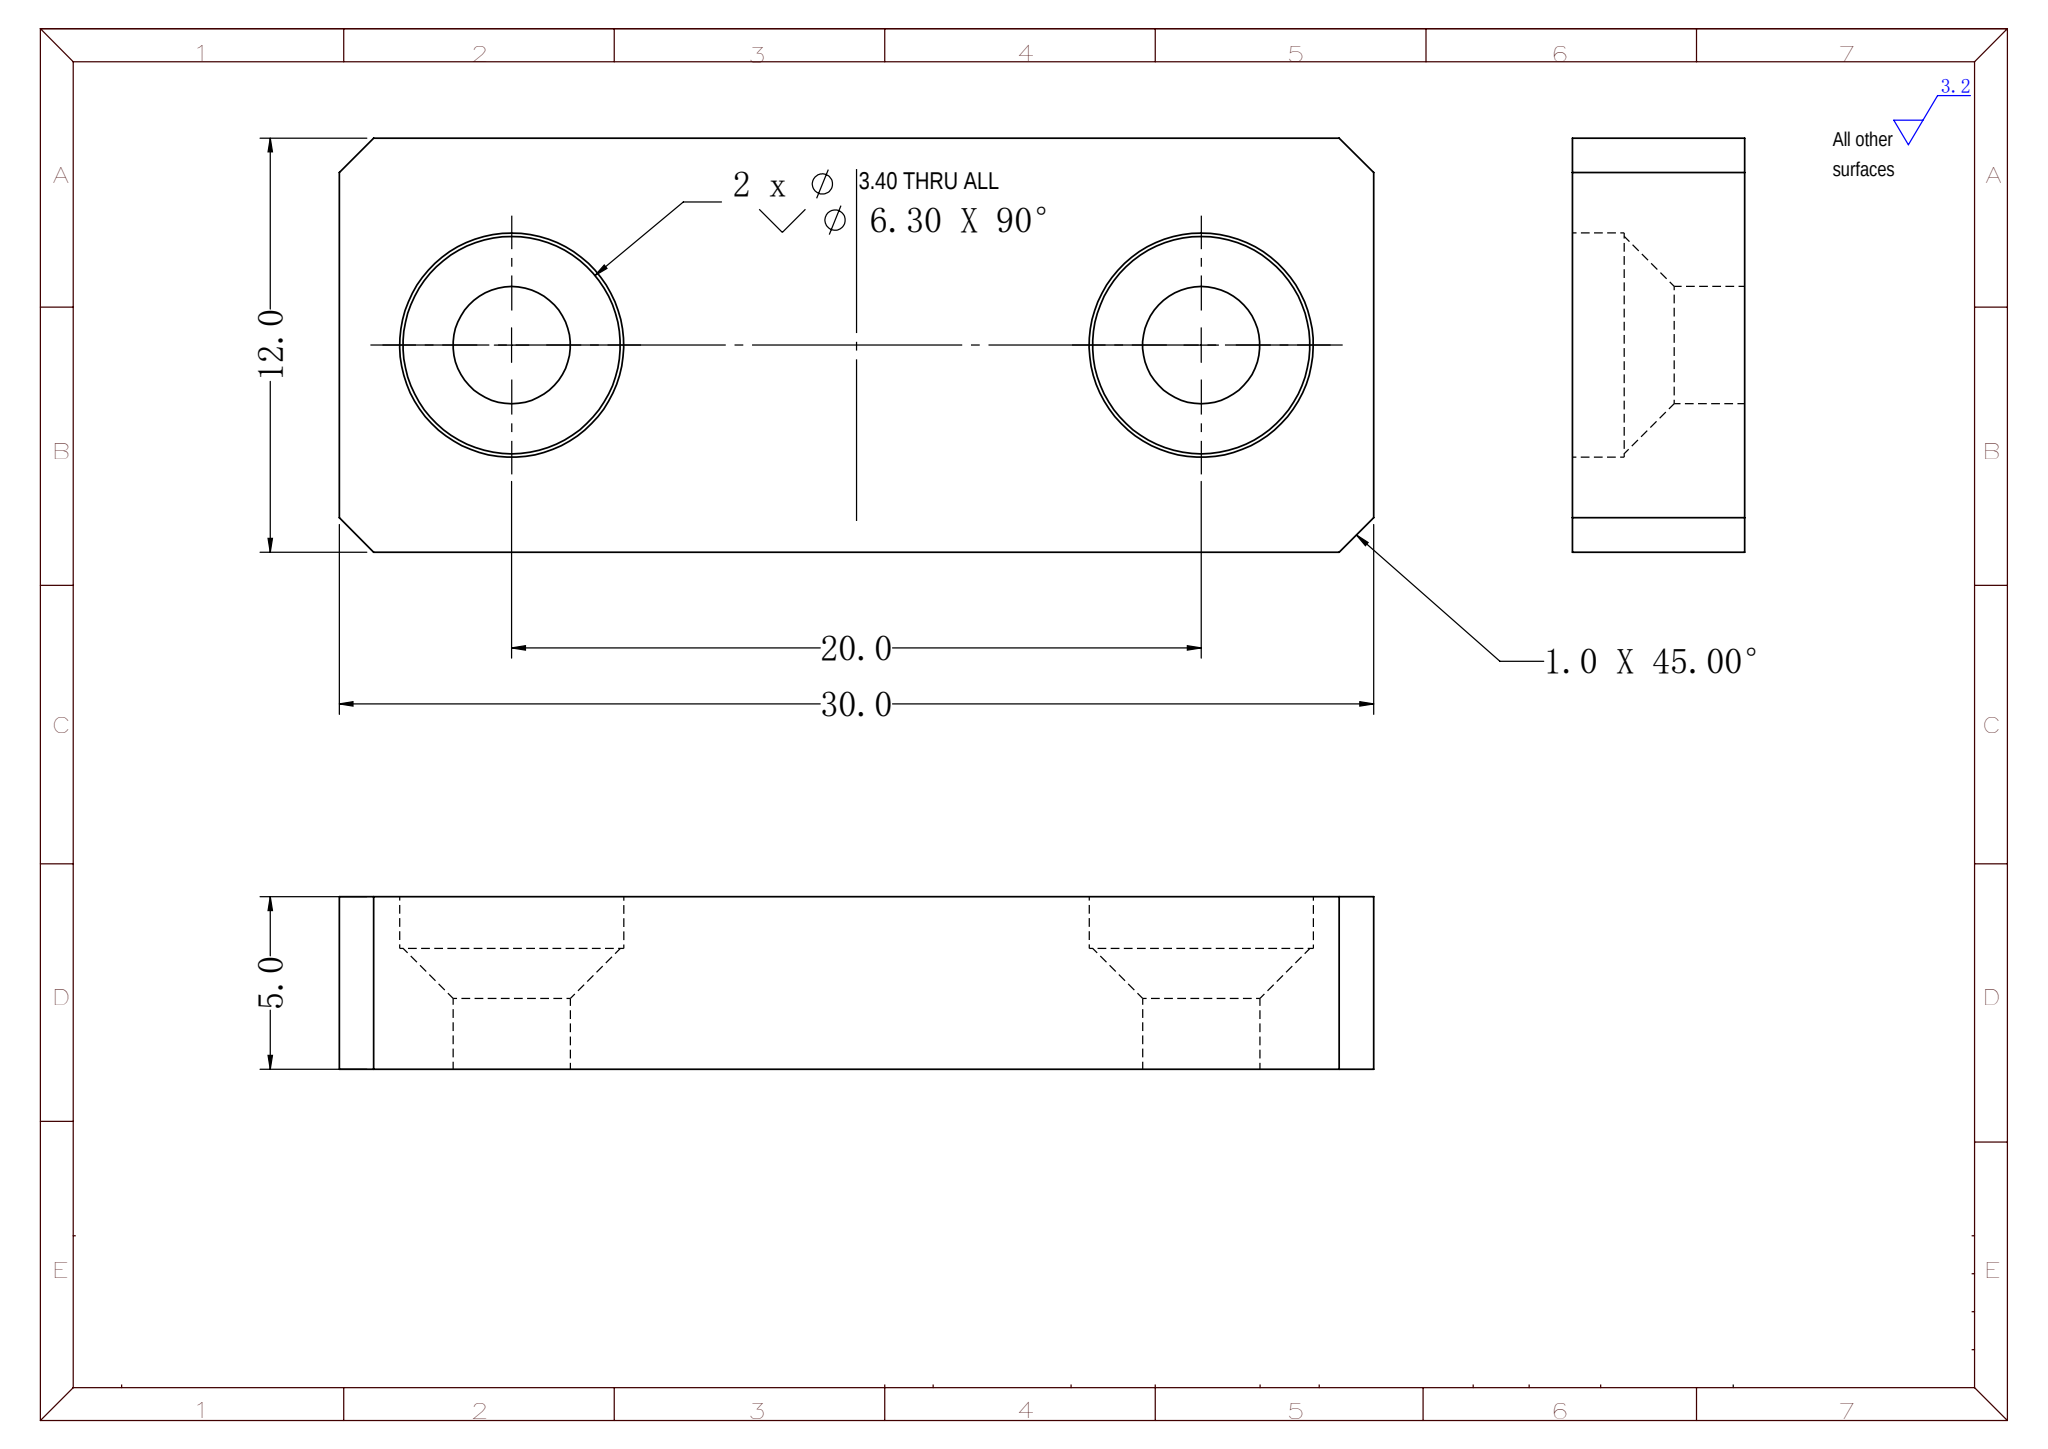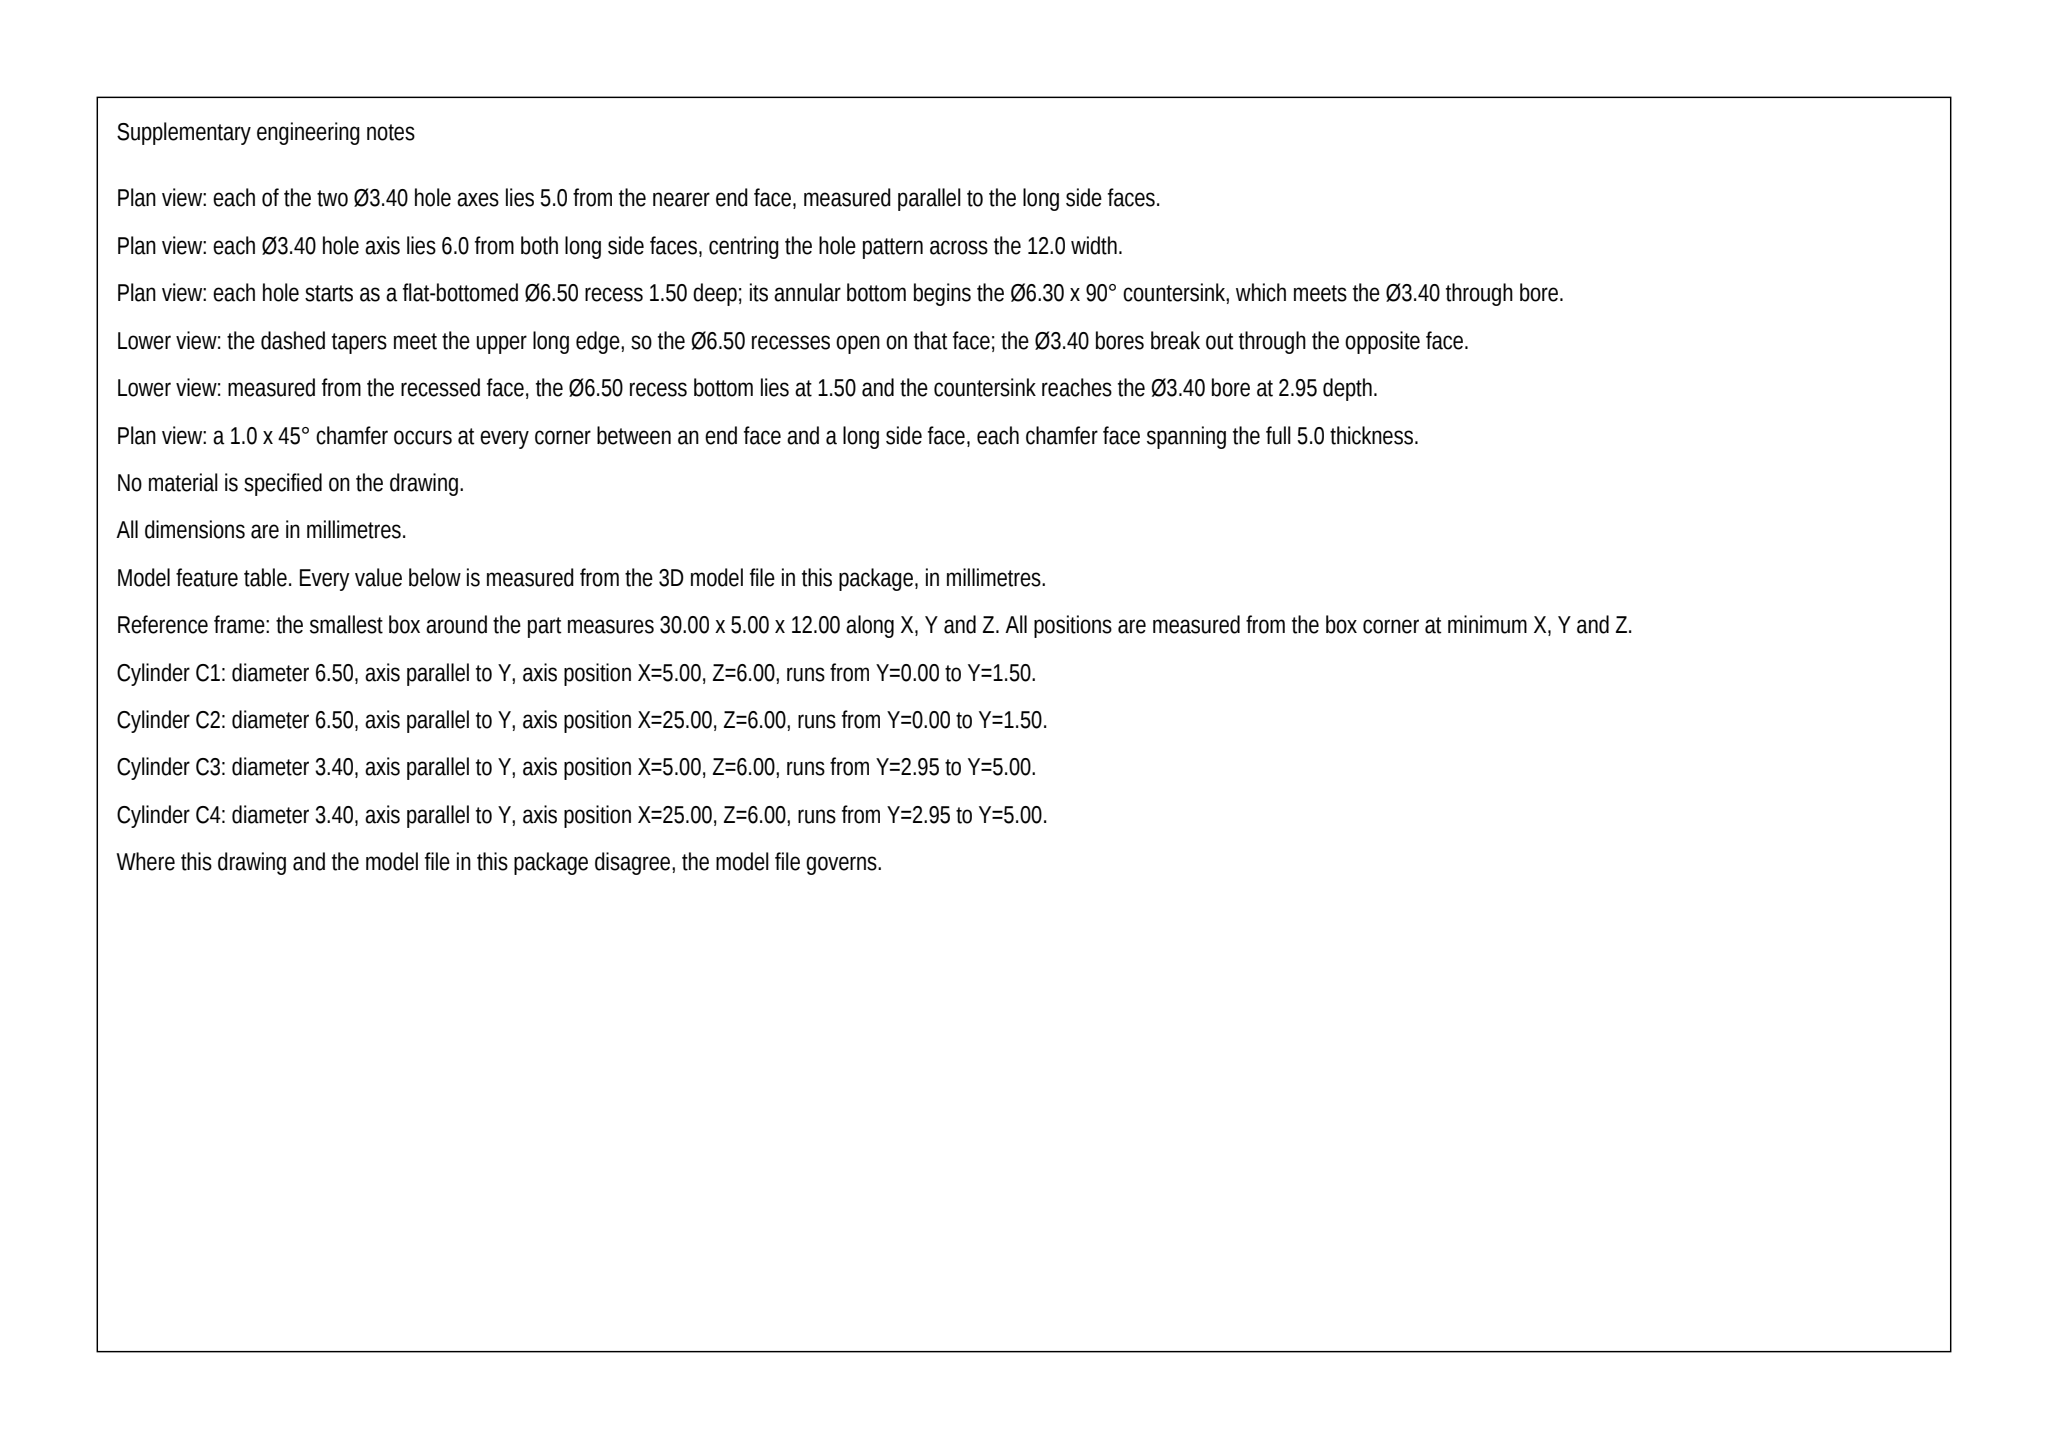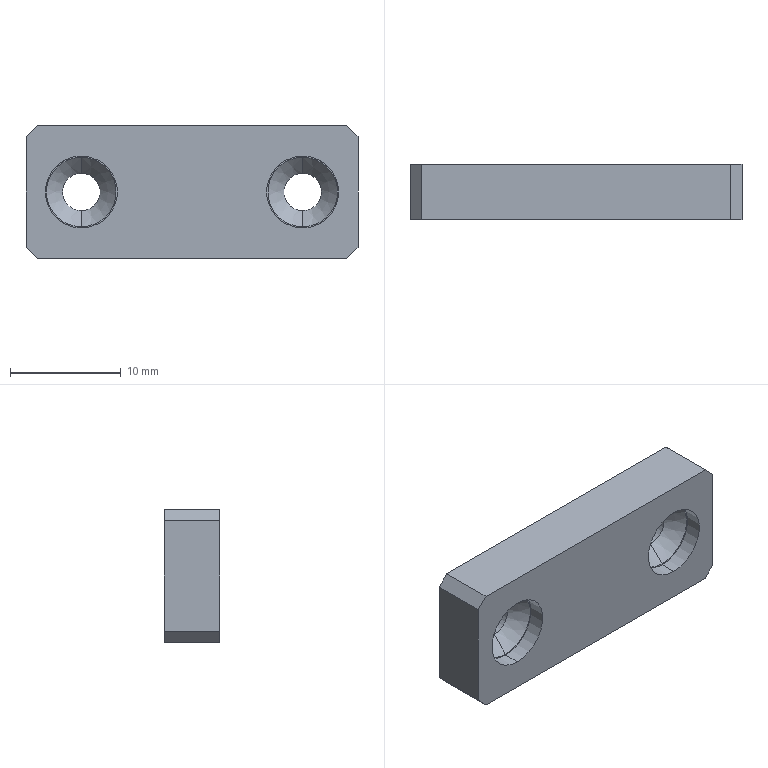Part | SolidWorks | mm | 1 solid | 24 faces | box 30 x 5 x 12 mm | volume 1598 mm3 | plane 12 | cylinder 8 | cone 4 | commonest cylinder face diameters 3.4 x4 6.5 x4
Drawing notes:
2 x CBORE Ø 6.50 DP 1.50 | from the solid: cylinders dia 6.5, axis y, len 1.5 at x=5 and x=25, z=6; y-plane at 1.5
1.0 X 45.00° CHAMFER, 4X | from the solid: four 45° corner chamfers on 30.0 x 12.0 outline, 1.0 leg each
build123d program:
from build123d import *

# Parameters (mm, degrees)
SKETCH1_W                                            = 30
SKETCH1_H                                            = 12
BOSS_EXTRUDE1_DEPTH                                  = 5
SKETCH4_R                                            = 3.25
CUT_EXTRUDE1_DEPTH                                   = 1.5
COUNTERSUNK_HOLE_1_FOR_M3_COUNTERSUNK_HE_D           = 3.4
COUNTERSUNK_HOLE_1_FOR_M3_COUNTERSUNK_HE_CSINK_D     = 6.3
COUNTERSUNK_HOLE_1_FOR_M3_COUNTERSUNK_HE_CSINK_ANGLE = 90
CHAMFER1_SIZE                                        = 1


with BuildPart() as part:
    # Sketch1 → Boss-Extrude1 (new body)
    with BuildSketch(Plane(origin=(0, 0, 0), x_dir=(1, 0, 0), z_dir=(0, 1, 0))):
        Rectangle(SKETCH1_W, SKETCH1_H)
    extrude(amount=BOSS_EXTRUDE1_DEPTH)

    # Sketch4 → Cut-Extrude1 (cut)
    with BuildSketch(Plane.XZ):
        with Locations(Location((10, 0, 0), (0, 0, 270))):
            Circle(SKETCH4_R)
        with Locations(Location((-10, 0, 0), (0, 0, 270))):
            Circle(SKETCH4_R)
    extrude(amount=-CUT_EXTRUDE1_DEPTH, mode=Mode.SUBTRACT)

    # Countersunk Hole 1 for M3 Countersunk He (through all)
    with Locations(Plane(origin=(10, 1.5, 0), x_dir=(0, 0, -1), z_dir=(0, -1, 0))):
        with Locations((0, 0), (0, -20)):
            CounterSinkHole(COUNTERSUNK_HOLE_1_FOR_M3_COUNTERSUNK_HE_D / 2, COUNTERSUNK_HOLE_1_FOR_M3_COUNTERSUNK_HE_CSINK_D / 2, counter_sink_angle=COUNTERSUNK_HOLE_1_FOR_M3_COUNTERSUNK_HE_CSINK_ANGLE)

    # Chamfer1
    chamfer1_edges = [part.edges().sort_by_distance(p)[0] for p in [
        (15, 2.5, 6),
        (-15, 2.5, 6),
        (-15, 2.5, -6),
        (15, 2.5, -6),
    ]]
    chamfer(chamfer1_edges, length=CHAMFER1_SIZE)


solid = part.part
STEP:
#1=CARTESIAN_POINT('',(10.,2.95,1.7));
#2=VERTEX_POINT('',#1);
#3=CARTESIAN_POINT('',(10.,2.95,-1.7));
#4=VERTEX_POINT('',#3);
#5=CARTESIAN_POINT('',(10.,2.95,0.));
#6=DIRECTION('',(0.,-1.,0.));
#7=DIRECTION('',(0.,0.,-1.));
#8=AXIS2_PLACEMENT_3D('',#5,#6,#7);
#9=CIRCLE('',#8,1.7);
#10=EDGE_CURVE('',#2,#4,#9,.T.);
#11=ORIENTED_EDGE('',*,*,#10,.F.);
#12=CARTESIAN_POINT('',(10.,1.5,3.15));
#13=VERTEX_POINT('',#12);
#14=CARTESIAN_POINT('',(10.,1.5,3.15));
#15=DIRECTION('',(0.,-0.7071,0.7071));
#16=VECTOR('',#15,1000.);
#17=LINE('',#14,#16);
#18=EDGE_CURVE('',#2,#13,#17,.T.);
#19=ORIENTED_EDGE('',*,*,#18,.T.);
#20=CARTESIAN_POINT('',(10.,1.5,-3.15));
#21=VERTEX_POINT('',#20);
#22=CARTESIAN_POINT('',(10.,1.5,0.));
#23=DIRECTION('',(0.,-1.,0.));
#24=DIRECTION('',(0.,0.,-1.));
#25=AXIS2_PLACEMENT_3D('',#22,#23,#24);
#26=CIRCLE('',#25,3.15);
#27=EDGE_CURVE('',#13,#21,#26,.T.);
#28=ORIENTED_EDGE('',*,*,#27,.T.);
#29=CARTESIAN_POINT('',(10.,1.5,-3.15));
#30=DIRECTION('',(0.,-0.7071,-0.7071));
#31=VECTOR('',#30,1000.);
#32=LINE('',#29,#31);
#33=EDGE_CURVE('',#4,#21,#32,.T.);
#34=ORIENTED_EDGE('',*,*,#33,.F.);
#35=EDGE_LOOP('',(#11,#19,#28,#34));
#36=FACE_OUTER_BOUND('',#35,.T.);
#37=CARTESIAN_POINT('',(10.,1.5,0.));
#38=DIRECTION('',(0.,-1.,0.));
#39=DIRECTION('',(0.,0.,-1.));
#40=AXIS2_PLACEMENT_3D('',#37,#38,#39);
#41=CONICAL_SURFACE('',#40,3.15,0.7854);
#42=ADVANCED_FACE('',(#36),#41,.F.);
#43=CARTESIAN_POINT('',(10.,5.,1.7));
#44=VERTEX_POINT('',#43);
#45=CARTESIAN_POINT('',(10.,5.,-1.7));
#46=VERTEX_POINT('',#45);
#47=CARTESIAN_POINT('',(10.,5.,0.));
#48=DIRECTION('',(0.,-1.,0.));
#49=DIRECTION('',(0.,0.,-1.));
#50=AXIS2_PLACEMENT_3D('',#47,#48,#49);
#51=CIRCLE('',#50,1.7);
#52=EDGE_CURVE('',#44,#46,#51,.T.);
#53=ORIENTED_EDGE('',*,*,#52,.F.);
#54=CARTESIAN_POINT('',(10.,1.5,1.7));
#55=DIRECTION('',(0.,-1.,0.));
#56=VECTOR('',#55,1000.);
#57=LINE('',#54,#56);
#58=EDGE_CURVE('',#44,#2,#57,.T.);
#59=ORIENTED_EDGE('',*,*,#58,.T.);
#60=ORIENTED_EDGE('',*,*,#10,.T.);
#61=CARTESIAN_POINT('',(10.,1.5,-1.7));
#62=DIRECTION('',(0.,-1.,0.));
#63=VECTOR('',#62,1000.);
#64=LINE('',#61,#63);
#65=EDGE_CURVE('',#46,#4,#64,.T.);
#66=ORIENTED_EDGE('',*,*,#65,.F.);
#67=EDGE_LOOP('',(#53,#59,#60,#66));
#68=FACE_OUTER_BOUND('',#67,.T.);
#69=CARTESIAN_POINT('',(10.,1.5,0.));
#70=DIRECTION('',(0.,-1.,0.));
#71=DIRECTION('',(0.,0.,-1.));
#72=AXIS2_PLACEMENT_3D('',#69,#70,#71);
#73=CYLINDRICAL_SURFACE('',#72,1.7);
#74=ADVANCED_FACE('',(#68),#73,.F.);
#75=CARTESIAN_POINT('',(-10.,2.95,1.7));
#76=VERTEX_POINT('',#75);
#77=CARTESIAN_POINT('',(-10.,2.95,-1.7));
#78=VERTEX_POINT('',#77);
#79=CARTESIAN_POINT('',(-10.,2.95,-0.));
#80=DIRECTION('',(0.,-1.,0.));
#81=DIRECTION('',(0.,0.,-1.));
#82=AXIS2_PLACEMENT_3D('',#79,#80,#81);
#83=CIRCLE('',#82,1.7);
#84=EDGE_CURVE('',#76,#78,#83,.T.);
#85=ORIENTED_EDGE('',*,*,#84,.F.);
#86=CARTESIAN_POINT('',(-10.,1.5,3.15));
#87=VERTEX_POINT('',#86);
#88=CARTESIAN_POINT('',(-10.,1.5,3.15));
#89=DIRECTION('',(0.,-0.7071,0.7071));
#90=VECTOR('',#89,1000.);
#91=LINE('',#88,#90);
#92=EDGE_CURVE('',#76,#87,#91,.T.);
#93=ORIENTED_EDGE('',*,*,#92,.T.);
#94=CARTESIAN_POINT('',(-10.,1.5,-3.15));
#95=VERTEX_POINT('',#94);
#96=CARTESIAN_POINT('',(-10.,1.5,-0.));
#97=DIRECTION('',(0.,-1.,0.));
#98=DIRECTION('',(0.,0.,-1.));
#99=AXIS2_PLACEMENT_3D('',#96,#97,#98);
#100=CIRCLE('',#99,3.15);
#101=EDGE_CURVE('',#87,#95,#100,.T.);
#102=ORIENTED_EDGE('',*,*,#101,.T.);
#103=CARTESIAN_POINT('',(-10.,1.5,-3.15));
#104=DIRECTION('',(0.,-0.7071,-0.7071));
#105=VECTOR('',#104,1000.);
#106=LINE('',#103,#105);
#107=EDGE_CURVE('',#78,#95,#106,.T.);
#108=ORIENTED_EDGE('',*,*,#107,.F.);
#109=EDGE_LOOP('',(#85,#93,#102,#108));
#110=FACE_OUTER_BOUND('',#109,.T.);
#111=CARTESIAN_POINT('',(-10.,1.5,-0.));
#112=DIRECTION('',(0.,-1.,0.));
#113=DIRECTION('',(0.,0.,-1.));
#114=AXIS2_PLACEMENT_3D('',#111,#112,#113);
#115=CONICAL_SURFACE('',#114,3.15,0.7854);
#116=ADVANCED_FACE('',(#110),#115,.F.);
#117=CARTESIAN_POINT('',(-10.,5.,1.7));
#118=VERTEX_POINT('',#117);
#119=CARTESIAN_POINT('',(-10.,5.,-1.7));
#120=VERTEX_POINT('',#119);
#121=CARTESIAN_POINT('',(-10.,5.,-0.));
#122=DIRECTION('',(0.,-1.,0.));
#123=DIRECTION('',(0.,0.,-1.));
#124=AXIS2_PLACEMENT_3D('',#121,#122,#123);
#125=CIRCLE('',#124,1.7);
#126=EDGE_CURVE('',#118,#120,#125,.T.);
#127=ORIENTED_EDGE('',*,*,#126,.F.);
#128=CARTESIAN_POINT('',(-10.,1.5,1.7));
#129=DIRECTION('',(0.,-1.,0.));
#130=VECTOR('',#129,1000.);
#131=LINE('',#128,#130);
#132=EDGE_CURVE('',#118,#76,#131,.T.);
#133=ORIENTED_EDGE('',*,*,#132,.T.);
#134=ORIENTED_EDGE('',*,*,#84,.T.);
#135=CARTESIAN_POINT('',(-10.,1.5,-1.7));
#136=DIRECTION('',(0.,-1.,0.));
#137=VECTOR('',#136,1000.);
#138=LINE('',#135,#137);
#139=EDGE_CURVE('',#120,#78,#138,.T.);
#140=ORIENTED_EDGE('',*,*,#139,.F.);
#141=EDGE_LOOP('',(#127,#133,#134,#140));
#142=FACE_OUTER_BOUND('',#141,.T.);
#143=CARTESIAN_POINT('',(-10.,1.5,-0.));
#144=DIRECTION('',(0.,-1.,0.));
#145=DIRECTION('',(0.,0.,-1.));
#146=AXIS2_PLACEMENT_3D('',#143,#144,#145);
#147=CYLINDRICAL_SURFACE('',#146,1.7);
#148=ADVANCED_FACE('',(#142),#147,.F.);
#149=CARTESIAN_POINT('',(-10.,1.5,3.25));
#150=VERTEX_POINT('',#149);
#151=CARTESIAN_POINT('',(-10.,1.5,-3.25));
#152=VERTEX_POINT('',#151);
#153=CARTESIAN_POINT('',(-10.,1.5,-0.));
#154=DIRECTION('',(0.,-1.,0.));
#155=DIRECTION('',(0.,0.,-1.));
#156=AXIS2_PLACEMENT_3D('',#153,#154,#155);
#157=CIRCLE('',#156,3.25);
#158=EDGE_CURVE('',#150,#152,#157,.T.);
#159=ORIENTED_EDGE('',*,*,#158,.F.);
#160=CARTESIAN_POINT('',(-10.,0.,3.25));
#161=VERTEX_POINT('',#160);
#162=CARTESIAN_POINT('',(-10.,1.5,3.25));
#163=DIRECTION('',(0.,-1.,0.));
#164=VECTOR('',#163,1000.);
#165=LINE('',#162,#164);
#166=EDGE_CURVE('',#150,#161,#165,.T.);
#167=ORIENTED_EDGE('',*,*,#166,.T.);
#168=CARTESIAN_POINT('',(-10.,0.,-3.25));
#169=VERTEX_POINT('',#168);
#170=CARTESIAN_POINT('',(-10.,0.,-0.));
#171=DIRECTION('',(0.,-1.,0.));
#172=DIRECTION('',(0.,0.,-1.));
#173=AXIS2_PLACEMENT_3D('',#170,#171,#172);
#174=CIRCLE('',#173,3.25);
#175=EDGE_CURVE('',#161,#169,#174,.T.);
#176=ORIENTED_EDGE('',*,*,#175,.T.);
#177=CARTESIAN_POINT('',(-10.,1.5,-3.25));
#178=DIRECTION('',(0.,-1.,0.));
#179=VECTOR('',#178,1000.);
#180=LINE('',#177,#179);
#181=EDGE_CURVE('',#152,#169,#180,.T.);
#182=ORIENTED_EDGE('',*,*,#181,.F.);
#183=EDGE_LOOP('',(#159,#167,#176,#182));
#184=FACE_OUTER_BOUND('',#183,.T.);
#185=CARTESIAN_POINT('',(-10.,1.5,-0.));
#186=DIRECTION('',(0.,-1.,0.));
#187=DIRECTION('',(0.,0.,-1.));
#188=AXIS2_PLACEMENT_3D('',#185,#186,#187);
#189=CYLINDRICAL_SURFACE('',#188,3.25);
#190=ADVANCED_FACE('',(#184),#189,.F.);
#191=CARTESIAN_POINT('',(10.,1.5,3.25));
#192=VERTEX_POINT('',#191);
#193=CARTESIAN_POINT('',(10.,1.5,-3.25));
#194=VERTEX_POINT('',#193);
#195=CARTESIAN_POINT('',(10.,1.5,0.));
#196=DIRECTION('',(0.,-1.,0.));
#197=DIRECTION('',(0.,0.,-1.));
#198=AXIS2_PLACEMENT_3D('',#195,#196,#197);
#199=CIRCLE('',#198,3.25);
#200=EDGE_CURVE('',#192,#194,#199,.T.);
#201=ORIENTED_EDGE('',*,*,#200,.F.);
#202=CARTESIAN_POINT('',(10.,0.,3.25));
#203=VERTEX_POINT('',#202);
#204=CARTESIAN_POINT('',(10.,1.5,3.25));
#205=DIRECTION('',(0.,-1.,0.));
#206=VECTOR('',#205,1000.);
#207=LINE('',#204,#206);
#208=EDGE_CURVE('',#192,#203,#207,.T.);
#209=ORIENTED_EDGE('',*,*,#208,.T.);
#210=CARTESIAN_POINT('',(10.,0.,-3.25));
#211=VERTEX_POINT('',#210);
#212=CARTESIAN_POINT('',(10.,0.,0.));
#213=DIRECTION('',(0.,-1.,0.));
#214=DIRECTION('',(0.,0.,-1.));
#215=AXIS2_PLACEMENT_3D('',#212,#213,#214);
#216=CIRCLE('',#215,3.25);
#217=EDGE_CURVE('',#203,#211,#216,.T.);
#218=ORIENTED_EDGE('',*,*,#217,.T.);
#219=CARTESIAN_POINT('',(10.,1.5,-3.25));
#220=DIRECTION('',(0.,-1.,0.));
#221=VECTOR('',#220,1000.);
#222=LINE('',#219,#221);
#223=EDGE_CURVE('',#194,#211,#222,.T.);
#224=ORIENTED_EDGE('',*,*,#223,.F.);
#225=EDGE_LOOP('',(#201,#209,#218,#224));
#226=FACE_OUTER_BOUND('',#225,.T.);
#227=CARTESIAN_POINT('',(10.,1.5,0.));
#228=DIRECTION('',(0.,-1.,0.));
#229=DIRECTION('',(0.,0.,-1.));
#230=AXIS2_PLACEMENT_3D('',#227,#228,#229);
#231=CYLINDRICAL_SURFACE('',#230,3.25);
#232=ADVANCED_FACE('',(#226),#231,.F.);
#233=CARTESIAN_POINT('',(15.,0.,5.));
#234=VERTEX_POINT('',#233);
#235=CARTESIAN_POINT('',(15.,0.,-5.));
#236=VERTEX_POINT('',#235);
#237=CARTESIAN_POINT('',(15.,0.,-6.));
#238=DIRECTION('',(-0.,0.,-1.));
#239=VECTOR('',#238,1000.);
#240=LINE('',#237,#239);
#241=EDGE_CURVE('',#234,#236,#240,.T.);
#242=ORIENTED_EDGE('',*,*,#241,.T.);
#243=CARTESIAN_POINT('',(15.,5.,-5.));
#244=VERTEX_POINT('',#243);
#245=CARTESIAN_POINT('',(15.,5.,-5.));
#246=DIRECTION('',(0.,1.,0.));
#247=VECTOR('',#246,1000.);
#248=LINE('',#245,#247);
#249=EDGE_CURVE('',#236,#244,#248,.T.);
#250=ORIENTED_EDGE('',*,*,#249,.T.);
#251=CARTESIAN_POINT('',(15.,5.,5.));
#252=VERTEX_POINT('',#251);
#253=CARTESIAN_POINT('',(15.,5.,-6.));
#254=DIRECTION('',(-0.,0.,-1.));
#255=VECTOR('',#254,1000.);
#256=LINE('',#253,#255);
#257=EDGE_CURVE('',#252,#244,#256,.T.);
#258=ORIENTED_EDGE('',*,*,#257,.F.);
#259=CARTESIAN_POINT('',(15.,5.,5.));
#260=DIRECTION('',(0.,-1.,0.));
#261=VECTOR('',#260,1000.);
#262=LINE('',#259,#261);
#263=EDGE_CURVE('',#252,#234,#262,.T.);
#264=ORIENTED_EDGE('',*,*,#263,.T.);
#265=EDGE_LOOP('',(#242,#250,#258,#264));
#266=FACE_OUTER_BOUND('',#265,.T.);
#267=CARTESIAN_POINT('',(15.,5.,-6.));
#268=DIRECTION('',(-1.,0.,0.));
#269=DIRECTION('',(0.,0.,1.));
#270=AXIS2_PLACEMENT_3D('',#267,#268,#269);
#271=PLANE('',#270);
#272=ADVANCED_FACE('',(#266),#271,.F.);
#273=CARTESIAN_POINT('',(14.,5.,-6.));
#274=VERTEX_POINT('',#273);
#275=CARTESIAN_POINT('',(-14.,5.,-6.));
#276=VERTEX_POINT('',#275);
#277=CARTESIAN_POINT('',(-15.,5.,-6.));
#278=DIRECTION('',(-1.,0.,0.));
#279=VECTOR('',#278,1000.);
#280=LINE('',#277,#279);
#281=EDGE_CURVE('',#274,#276,#280,.T.);
#282=ORIENTED_EDGE('',*,*,#281,.F.);
#283=CARTESIAN_POINT('',(14.,0.,-6.));
#284=VERTEX_POINT('',#283);
#285=CARTESIAN_POINT('',(14.,5.,-6.));
#286=DIRECTION('',(0.,-1.,0.));
#287=VECTOR('',#286,1000.);
#288=LINE('',#285,#287);
#289=EDGE_CURVE('',#274,#284,#288,.T.);
#290=ORIENTED_EDGE('',*,*,#289,.T.);
#291=CARTESIAN_POINT('',(-14.,0.,-6.));
#292=VERTEX_POINT('',#291);
#293=CARTESIAN_POINT('',(-15.,0.,-6.));
#294=DIRECTION('',(-1.,0.,0.));
#295=VECTOR('',#294,1000.);
#296=LINE('',#293,#295);
#297=EDGE_CURVE('',#284,#292,#296,.T.);
#298=ORIENTED_EDGE('',*,*,#297,.T.);
#299=CARTESIAN_POINT('',(-14.,5.,-6.));
#300=DIRECTION('',(0.,1.,0.));
#301=VECTOR('',#300,1000.);
#302=LINE('',#299,#301);
#303=EDGE_CURVE('',#292,#276,#302,.T.);
#304=ORIENTED_EDGE('',*,*,#303,.T.);
#305=EDGE_LOOP('',(#282,#290,#298,#304));
#306=FACE_OUTER_BOUND('',#305,.T.);
#307=CARTESIAN_POINT('',(-15.,5.,-6.));
#308=DIRECTION('',(0.,0.,1.));
#309=DIRECTION('',(1.,0.,0.));
#310=AXIS2_PLACEMENT_3D('',#307,#308,#309);
#311=PLANE('',#310);
#312=ADVANCED_FACE('',(#306),#311,.F.);
#313=CARTESIAN_POINT('',(-15.,5.,-5.));
#314=VERTEX_POINT('',#313);
#315=CARTESIAN_POINT('',(-15.,5.,5.));
#316=VERTEX_POINT('',#315);
#317=CARTESIAN_POINT('',(-15.,5.,-6.));
#318=DIRECTION('',(0.,0.,1.));
#319=VECTOR('',#318,1000.);
#320=LINE('',#317,#319);
#321=EDGE_CURVE('',#314,#316,#320,.T.);
#322=ORIENTED_EDGE('',*,*,#321,.F.);
#323=CARTESIAN_POINT('',(-15.,0.,-5.));
#324=VERTEX_POINT('',#323);
#325=CARTESIAN_POINT('',(-15.,5.,-5.));
#326=DIRECTION('',(0.,-1.,0.));
#327=VECTOR('',#326,1000.);
#328=LINE('',#325,#327);
#329=EDGE_CURVE('',#314,#324,#328,.T.);
#330=ORIENTED_EDGE('',*,*,#329,.T.);
#331=CARTESIAN_POINT('',(-15.,0.,5.));
#332=VERTEX_POINT('',#331);
#333=CARTESIAN_POINT('',(-15.,0.,-6.));
#334=DIRECTION('',(0.,0.,1.));
#335=VECTOR('',#334,1000.);
#336=LINE('',#333,#335);
#337=EDGE_CURVE('',#324,#332,#336,.T.);
#338=ORIENTED_EDGE('',*,*,#337,.T.);
#339=CARTESIAN_POINT('',(-15.,5.,5.));
#340=DIRECTION('',(0.,1.,0.));
#341=VECTOR('',#340,1000.);
#342=LINE('',#339,#341);
#343=EDGE_CURVE('',#332,#316,#342,.T.);
#344=ORIENTED_EDGE('',*,*,#343,.T.);
#345=EDGE_LOOP('',(#322,#330,#338,#344));
#346=FACE_OUTER_BOUND('',#345,.T.);
#347=CARTESIAN_POINT('',(-15.,5.,-6.));
#348=DIRECTION('',(1.,0.,-0.));
#349=DIRECTION('',(-0.,0.,-1.));
#350=AXIS2_PLACEMENT_3D('',#347,#348,#349);
#351=PLANE('',#350);
#352=ADVANCED_FACE('',(#346),#351,.F.);
#353=CARTESIAN_POINT('',(-14.,0.,6.));
#354=VERTEX_POINT('',#353);
#355=CARTESIAN_POINT('',(14.,0.,6.));
#356=VERTEX_POINT('',#355);
#357=CARTESIAN_POINT('',(-15.,0.,6.));
#358=DIRECTION('',(1.,0.,0.));
#359=VECTOR('',#358,1000.);
#360=LINE('',#357,#359);
#361=EDGE_CURVE('',#354,#356,#360,.T.);
#362=ORIENTED_EDGE('',*,*,#361,.T.);
#363=CARTESIAN_POINT('',(14.,5.,6.));
#364=VERTEX_POINT('',#363);
#365=CARTESIAN_POINT('',(14.,5.,6.));
#366=DIRECTION('',(0.,1.,0.));
#367=VECTOR('',#366,1000.);
#368=LINE('',#365,#367);
#369=EDGE_CURVE('',#356,#364,#368,.T.);
#370=ORIENTED_EDGE('',*,*,#369,.T.);
#371=CARTESIAN_POINT('',(-14.,5.,6.));
#372=VERTEX_POINT('',#371);
#373=CARTESIAN_POINT('',(-15.,5.,6.));
#374=DIRECTION('',(1.,0.,0.));
#375=VECTOR('',#374,1000.);
#376=LINE('',#373,#375);
#377=EDGE_CURVE('',#372,#364,#376,.T.);
#378=ORIENTED_EDGE('',*,*,#377,.F.);
#379=CARTESIAN_POINT('',(-14.,5.,6.));
#380=DIRECTION('',(0.,-1.,0.));
#381=VECTOR('',#380,1000.);
#382=LINE('',#379,#381);
#383=EDGE_CURVE('',#372,#354,#382,.T.);
#384=ORIENTED_EDGE('',*,*,#383,.T.);
#385=EDGE_LOOP('',(#362,#370,#378,#384));
#386=FACE_OUTER_BOUND('',#385,.T.);
#387=CARTESIAN_POINT('',(-15.,5.,6.));
#388=DIRECTION('',(0.,0.,-1.));
#389=DIRECTION('',(-1.,0.,0.));
#390=AXIS2_PLACEMENT_3D('',#387,#388,#389);
#391=PLANE('',#390);
#392=ADVANCED_FACE('',(#386),#391,.F.);
#393=CARTESIAN_POINT('',(10.,5.,0.));
#394=DIRECTION('',(0.,-1.,0.));
#395=DIRECTION('',(0.,0.,-1.));
#396=AXIS2_PLACEMENT_3D('',#393,#394,#395);
#397=CIRCLE('',#396,1.7);
#398=EDGE_CURVE('',#46,#44,#397,.T.);
#399=ORIENTED_EDGE('',*,*,#398,.T.);
#400=ORIENTED_EDGE('',*,*,#52,.T.);
#401=EDGE_LOOP('',(#399,#400));
#402=FACE_BOUND('',#401,.T.);
#403=CARTESIAN_POINT('',(-10.,5.,-0.));
#404=DIRECTION('',(0.,-1.,0.));
#405=DIRECTION('',(0.,0.,-1.));
#406=AXIS2_PLACEMENT_3D('',#403,#404,#405);
#407=CIRCLE('',#406,1.7);
#408=EDGE_CURVE('',#120,#118,#407,.T.);
#409=ORIENTED_EDGE('',*,*,#408,.T.);
#410=ORIENTED_EDGE('',*,*,#126,.T.);
#411=EDGE_LOOP('',(#409,#410));
#412=FACE_BOUND('',#411,.T.);
#413=ORIENTED_EDGE('',*,*,#257,.T.);
#414=CARTESIAN_POINT('',(10.,5.,-10.));
#415=DIRECTION('',(-0.7071,0.,-0.7071));
#416=VECTOR('',#415,1000.);
#417=LINE('',#414,#416);
#418=EDGE_CURVE('',#244,#274,#417,.T.);
#419=ORIENTED_EDGE('',*,*,#418,.T.);
#420=ORIENTED_EDGE('',*,*,#281,.T.);
#421=CARTESIAN_POINT('',(-10.,5.,-10.));
#422=DIRECTION('',(-0.7071,0.,0.7071));
#423=VECTOR('',#422,1000.);
#424=LINE('',#421,#423);
#425=EDGE_CURVE('',#276,#314,#424,.T.);
#426=ORIENTED_EDGE('',*,*,#425,.T.);
#427=ORIENTED_EDGE('',*,*,#321,.T.);
#428=CARTESIAN_POINT('',(-10.,5.,10.));
#429=DIRECTION('',(0.7071,0.,0.7071));
#430=VECTOR('',#429,1000.);
#431=LINE('',#428,#430);
#432=EDGE_CURVE('',#316,#372,#431,.T.);
#433=ORIENTED_EDGE('',*,*,#432,.T.);
#434=ORIENTED_EDGE('',*,*,#377,.T.);
#435=CARTESIAN_POINT('',(10.,5.,10.));
#436=DIRECTION('',(0.7071,0.,-0.7071));
#437=VECTOR('',#436,1000.);
#438=LINE('',#435,#437);
#439=EDGE_CURVE('',#364,#252,#438,.T.);
#440=ORIENTED_EDGE('',*,*,#439,.T.);
#441=EDGE_LOOP('',(#413,#419,#420,#426,#427,#433,#434,#440));
#442=FACE_OUTER_BOUND('',#441,.T.);
#443=CARTESIAN_POINT('',(0.,5.,0.));
#444=DIRECTION('',(0.,1.,0.));
#445=DIRECTION('',(0.,0.,1.));
#446=AXIS2_PLACEMENT_3D('',#443,#444,#445);
#447=PLANE('',#446);
#448=ADVANCED_FACE('',(#402,#412,#442),#447,.T.);
#449=CARTESIAN_POINT('',(-10.,0.,-0.));
#450=DIRECTION('',(0.,-1.,0.));
#451=DIRECTION('',(0.,0.,-1.));
#452=AXIS2_PLACEMENT_3D('',#449,#450,#451);
#453=CIRCLE('',#452,3.25);
#454=EDGE_CURVE('',#169,#161,#453,.T.);
#455=ORIENTED_EDGE('',*,*,#454,.F.);
#456=ORIENTED_EDGE('',*,*,#175,.F.);
#457=EDGE_LOOP('',(#455,#456));
#458=FACE_BOUND('',#457,.T.);
#459=CARTESIAN_POINT('',(10.,0.,0.));
#460=DIRECTION('',(0.,-1.,0.));
#461=DIRECTION('',(0.,0.,-1.));
#462=AXIS2_PLACEMENT_3D('',#459,#460,#461);
#463=CIRCLE('',#462,3.25);
#464=EDGE_CURVE('',#211,#203,#463,.T.);
#465=ORIENTED_EDGE('',*,*,#464,.F.);
#466=ORIENTED_EDGE('',*,*,#217,.F.);
#467=EDGE_LOOP('',(#465,#466));
#468=FACE_BOUND('',#467,.T.);
#469=ORIENTED_EDGE('',*,*,#297,.F.);
#470=CARTESIAN_POINT('',(14.,0.,-6.));
#471=DIRECTION('',(0.7071,0.,0.7071));
#472=VECTOR('',#471,1000.);
#473=LINE('',#470,#472);
#474=EDGE_CURVE('',#284,#236,#473,.T.);
#475=ORIENTED_EDGE('',*,*,#474,.T.);
#476=ORIENTED_EDGE('',*,*,#241,.F.);
#477=CARTESIAN_POINT('',(15.,0.,5.));
#478=DIRECTION('',(-0.7071,0.,0.7071));
#479=VECTOR('',#478,1000.);
#480=LINE('',#477,#479);
#481=EDGE_CURVE('',#234,#356,#480,.T.);
#482=ORIENTED_EDGE('',*,*,#481,.T.);
#483=ORIENTED_EDGE('',*,*,#361,.F.);
#484=CARTESIAN_POINT('',(-14.,0.,6.));
#485=DIRECTION('',(-0.7071,0.,-0.7071));
#486=VECTOR('',#485,1000.);
#487=LINE('',#484,#486);
#488=EDGE_CURVE('',#354,#332,#487,.T.);
#489=ORIENTED_EDGE('',*,*,#488,.T.);
#490=ORIENTED_EDGE('',*,*,#337,.F.);
#491=CARTESIAN_POINT('',(-15.,0.,-5.));
#492=DIRECTION('',(0.7071,0.,-0.7071));
#493=VECTOR('',#492,1000.);
#494=LINE('',#491,#493);
#495=EDGE_CURVE('',#324,#292,#494,.T.);
#496=ORIENTED_EDGE('',*,*,#495,.T.);
#497=EDGE_LOOP('',(#469,#475,#476,#482,#483,#489,#490,#496));
#498=FACE_OUTER_BOUND('',#497,.T.);
#499=CARTESIAN_POINT('',(0.,0.,0.));
#500=DIRECTION('',(0.,1.,0.));
#501=DIRECTION('',(0.,0.,1.));
#502=AXIS2_PLACEMENT_3D('',#499,#500,#501);
#503=PLANE('',#502);
#504=ADVANCED_FACE('',(#458,#468,#498),#503,.F.);
#505=ORIENTED_EDGE('',*,*,#208,.F.);
#506=CARTESIAN_POINT('',(10.,1.5,0.));
#507=DIRECTION('',(0.,-1.,0.));
#508=DIRECTION('',(0.,0.,-1.));
#509=AXIS2_PLACEMENT_3D('',#506,#507,#508);
#510=CIRCLE('',#509,3.25);
#511=EDGE_CURVE('',#194,#192,#510,.T.);
#512=ORIENTED_EDGE('',*,*,#511,.F.);
#513=ORIENTED_EDGE('',*,*,#223,.T.);
#514=ORIENTED_EDGE('',*,*,#464,.T.);
#515=EDGE_LOOP('',(#505,#512,#513,#514));
#516=FACE_OUTER_BOUND('',#515,.T.);
#517=CARTESIAN_POINT('',(10.,1.5,0.));
#518=DIRECTION('',(0.,-1.,0.));
#519=DIRECTION('',(0.,0.,-1.));
#520=AXIS2_PLACEMENT_3D('',#517,#518,#519);
#521=CYLINDRICAL_SURFACE('',#520,3.25);
#522=ADVANCED_FACE('',(#516),#521,.F.);
#523=CARTESIAN_POINT('',(10.,1.5,0.));
#524=DIRECTION('',(0.,-1.,0.));
#525=DIRECTION('',(0.,0.,-1.));
#526=AXIS2_PLACEMENT_3D('',#523,#524,#525);
#527=CIRCLE('',#526,3.15);
#528=EDGE_CURVE('',#21,#13,#527,.T.);
#529=ORIENTED_EDGE('',*,*,#528,.F.);
#530=ORIENTED_EDGE('',*,*,#27,.F.);
#531=EDGE_LOOP('',(#529,#530));
#532=FACE_BOUND('',#531,.T.);
#533=ORIENTED_EDGE('',*,*,#511,.T.);
#534=ORIENTED_EDGE('',*,*,#200,.T.);
#535=EDGE_LOOP('',(#533,#534));
#536=FACE_OUTER_BOUND('',#535,.T.);
#537=CARTESIAN_POINT('',(10.,1.5,0.));
#538=DIRECTION('',(0.,-1.,0.));
#539=DIRECTION('',(0.,0.,-1.));
#540=AXIS2_PLACEMENT_3D('',#537,#538,#539);
#541=PLANE('',#540);
#542=ADVANCED_FACE('',(#532,#536),#541,.T.);
#543=ORIENTED_EDGE('',*,*,#166,.F.);
#544=CARTESIAN_POINT('',(-10.,1.5,-0.));
#545=DIRECTION('',(0.,-1.,0.));
#546=DIRECTION('',(0.,0.,-1.));
#547=AXIS2_PLACEMENT_3D('',#544,#545,#546);
#548=CIRCLE('',#547,3.25);
#549=EDGE_CURVE('',#152,#150,#548,.T.);
#550=ORIENTED_EDGE('',*,*,#549,.F.);
#551=ORIENTED_EDGE('',*,*,#181,.T.);
#552=ORIENTED_EDGE('',*,*,#454,.T.);
#553=EDGE_LOOP('',(#543,#550,#551,#552));
#554=FACE_OUTER_BOUND('',#553,.T.);
#555=CARTESIAN_POINT('',(-10.,1.5,-0.));
#556=DIRECTION('',(0.,-1.,0.));
#557=DIRECTION('',(0.,0.,-1.));
#558=AXIS2_PLACEMENT_3D('',#555,#556,#557);
#559=CYLINDRICAL_SURFACE('',#558,3.25);
#560=ADVANCED_FACE('',(#554),#559,.F.);
#561=CARTESIAN_POINT('',(-10.,1.5,-0.));
#562=DIRECTION('',(0.,-1.,0.));
#563=DIRECTION('',(0.,0.,-1.));
#564=AXIS2_PLACEMENT_3D('',#561,#562,#563);
#565=CIRCLE('',#564,3.15);
#566=EDGE_CURVE('',#95,#87,#565,.T.);
#567=ORIENTED_EDGE('',*,*,#566,.F.);
#568=ORIENTED_EDGE('',*,*,#101,.F.);
#569=EDGE_LOOP('',(#567,#568));
#570=FACE_BOUND('',#569,.T.);
#571=ORIENTED_EDGE('',*,*,#549,.T.);
#572=ORIENTED_EDGE('',*,*,#158,.T.);
#573=EDGE_LOOP('',(#571,#572));
#574=FACE_OUTER_BOUND('',#573,.T.);
#575=CARTESIAN_POINT('',(-10.,1.5,-0.));
#576=DIRECTION('',(0.,-1.,0.));
#577=DIRECTION('',(0.,0.,-1.));
#578=AXIS2_PLACEMENT_3D('',#575,#576,#577);
#579=PLANE('',#578);
#580=ADVANCED_FACE('',(#570,#574),#579,.T.);
#581=ORIENTED_EDGE('',*,*,#132,.F.);
#582=ORIENTED_EDGE('',*,*,#408,.F.);
#583=ORIENTED_EDGE('',*,*,#139,.T.);
#584=CARTESIAN_POINT('',(-10.,2.95,-0.));
#585=DIRECTION('',(0.,-1.,0.));
#586=DIRECTION('',(0.,0.,-1.));
#587=AXIS2_PLACEMENT_3D('',#584,#585,#586);
#588=CIRCLE('',#587,1.7);
#589=EDGE_CURVE('',#78,#76,#588,.T.);
#590=ORIENTED_EDGE('',*,*,#589,.T.);
#591=EDGE_LOOP('',(#581,#582,#583,#590));
#592=FACE_OUTER_BOUND('',#591,.T.);
#593=CARTESIAN_POINT('',(-10.,1.5,-0.));
#594=DIRECTION('',(0.,-1.,0.));
#595=DIRECTION('',(0.,0.,-1.));
#596=AXIS2_PLACEMENT_3D('',#593,#594,#595);
#597=CYLINDRICAL_SURFACE('',#596,1.7);
#598=ADVANCED_FACE('',(#592),#597,.F.);
#599=ORIENTED_EDGE('',*,*,#92,.F.);
#600=ORIENTED_EDGE('',*,*,#589,.F.);
#601=ORIENTED_EDGE('',*,*,#107,.T.);
#602=ORIENTED_EDGE('',*,*,#566,.T.);
#603=EDGE_LOOP('',(#599,#600,#601,#602));
#604=FACE_OUTER_BOUND('',#603,.T.);
#605=CARTESIAN_POINT('',(-10.,1.5,-0.));
#606=DIRECTION('',(0.,-1.,0.));
#607=DIRECTION('',(0.,0.,-1.));
#608=AXIS2_PLACEMENT_3D('',#605,#606,#607);
#609=CONICAL_SURFACE('',#608,3.15,0.7854);
#610=ADVANCED_FACE('',(#604),#609,.F.);
#611=ORIENTED_EDGE('',*,*,#58,.F.);
#612=ORIENTED_EDGE('',*,*,#398,.F.);
#613=ORIENTED_EDGE('',*,*,#65,.T.);
#614=CARTESIAN_POINT('',(10.,2.95,0.));
#615=DIRECTION('',(0.,-1.,0.));
#616=DIRECTION('',(0.,0.,-1.));
#617=AXIS2_PLACEMENT_3D('',#614,#615,#616);
#618=CIRCLE('',#617,1.7);
#619=EDGE_CURVE('',#4,#2,#618,.T.);
#620=ORIENTED_EDGE('',*,*,#619,.T.);
#621=EDGE_LOOP('',(#611,#612,#613,#620));
#622=FACE_OUTER_BOUND('',#621,.T.);
#623=CARTESIAN_POINT('',(10.,1.5,0.));
#624=DIRECTION('',(0.,-1.,0.));
#625=DIRECTION('',(0.,0.,-1.));
#626=AXIS2_PLACEMENT_3D('',#623,#624,#625);
#627=CYLINDRICAL_SURFACE('',#626,1.7);
#628=ADVANCED_FACE('',(#622),#627,.F.);
#629=ORIENTED_EDGE('',*,*,#18,.F.);
#630=ORIENTED_EDGE('',*,*,#619,.F.);
#631=ORIENTED_EDGE('',*,*,#33,.T.);
#632=ORIENTED_EDGE('',*,*,#528,.T.);
#633=EDGE_LOOP('',(#629,#630,#631,#632));
#634=FACE_OUTER_BOUND('',#633,.T.);
#635=CARTESIAN_POINT('',(10.,1.5,0.));
#636=DIRECTION('',(0.,-1.,0.));
#637=DIRECTION('',(0.,0.,-1.));
#638=AXIS2_PLACEMENT_3D('',#635,#636,#637);
#639=CONICAL_SURFACE('',#638,3.15,0.7854);
#640=ADVANCED_FACE('',(#634),#639,.F.);
#641=ORIENTED_EDGE('',*,*,#418,.F.);
#642=ORIENTED_EDGE('',*,*,#249,.F.);
#643=ORIENTED_EDGE('',*,*,#474,.F.);
#644=ORIENTED_EDGE('',*,*,#289,.F.);
#645=EDGE_LOOP('',(#641,#642,#643,#644));
#646=FACE_OUTER_BOUND('',#645,.T.);
#647=CARTESIAN_POINT('',(14.,5.,-6.));
#648=DIRECTION('',(-0.7071,0.,0.7071));
#649=DIRECTION('',(0.,-1.,0.));
#650=AXIS2_PLACEMENT_3D('',#647,#648,#649);
#651=PLANE('',#650);
#652=ADVANCED_FACE('',(#646),#651,.F.);
#653=ORIENTED_EDGE('',*,*,#439,.F.);
#654=ORIENTED_EDGE('',*,*,#369,.F.);
#655=ORIENTED_EDGE('',*,*,#481,.F.);
#656=ORIENTED_EDGE('',*,*,#263,.F.);
#657=EDGE_LOOP('',(#653,#654,#655,#656));
#658=FACE_OUTER_BOUND('',#657,.T.);
#659=CARTESIAN_POINT('',(15.,5.,5.));
#660=DIRECTION('',(-0.7071,0.,-0.7071));
#661=DIRECTION('',(0.,-1.,0.));
#662=AXIS2_PLACEMENT_3D('',#659,#660,#661);
#663=PLANE('',#662);
#664=ADVANCED_FACE('',(#658),#663,.F.);
#665=ORIENTED_EDGE('',*,*,#425,.F.);
#666=ORIENTED_EDGE('',*,*,#303,.F.);
#667=ORIENTED_EDGE('',*,*,#495,.F.);
#668=ORIENTED_EDGE('',*,*,#329,.F.);
#669=EDGE_LOOP('',(#665,#666,#667,#668));
#670=FACE_OUTER_BOUND('',#669,.T.);
#671=CARTESIAN_POINT('',(-15.,5.,-5.));
#672=DIRECTION('',(0.7071,0.,0.7071));
#673=DIRECTION('',(0.,-1.,0.));
#674=AXIS2_PLACEMENT_3D('',#671,#672,#673);
#675=PLANE('',#674);
#676=ADVANCED_FACE('',(#670),#675,.F.);
#677=ORIENTED_EDGE('',*,*,#432,.F.);
#678=ORIENTED_EDGE('',*,*,#343,.F.);
#679=ORIENTED_EDGE('',*,*,#488,.F.);
#680=ORIENTED_EDGE('',*,*,#383,.F.);
#681=EDGE_LOOP('',(#677,#678,#679,#680));
#682=FACE_OUTER_BOUND('',#681,.T.);
#683=CARTESIAN_POINT('',(-14.,5.,6.));
#684=DIRECTION('',(0.7071,0.,-0.7071));
#685=DIRECTION('',(0.,-1.,0.));
#686=AXIS2_PLACEMENT_3D('',#683,#684,#685);
#687=PLANE('',#686);
#688=ADVANCED_FACE('',(#682),#687,.F.);
#689=CLOSED_SHELL('',(#42,#74,#116,#148,#190,#232,#272,#312,#352,#392,#448,#504,#522,#542,#560,#580,#598,#610,#628,#640,#652,#664,#676,#688));
#690=MANIFOLD_SOLID_BREP('',#689);
#691=CARTESIAN_POINT('',(0.,0.,0.));
#692=DIRECTION('',(0.,0.,1.));
#693=DIRECTION('',(1.,0.,0.));
#694=AXIS2_PLACEMENT_3D('',#691,#692,#693);
#695=(LENGTH_UNIT()NAMED_UNIT(*)SI_UNIT(.MILLI.,.METRE.));
#696=UNCERTAINTY_MEASURE_WITH_UNIT(LENGTH_MEASURE(0.00001),#695,'','');
#697=(NAMED_UNIT(*)PLANE_ANGLE_UNIT()SI_UNIT($,.RADIAN.));
#698=(NAMED_UNIT(*)SI_UNIT($,.STERADIAN.)SOLID_ANGLE_UNIT());
#699=(GEOMETRIC_REPRESENTATION_CONTEXT(3)GLOBAL_UNCERTAINTY_ASSIGNED_CONTEXT((#696))GLOBAL_UNIT_ASSIGNED_CONTEXT((#695,#697,#698))REPRESENTATION_CONTEXT('',''));
#700=ADVANCED_BREP_SHAPE_REPRESENTATION('',(#690,#694),#699);